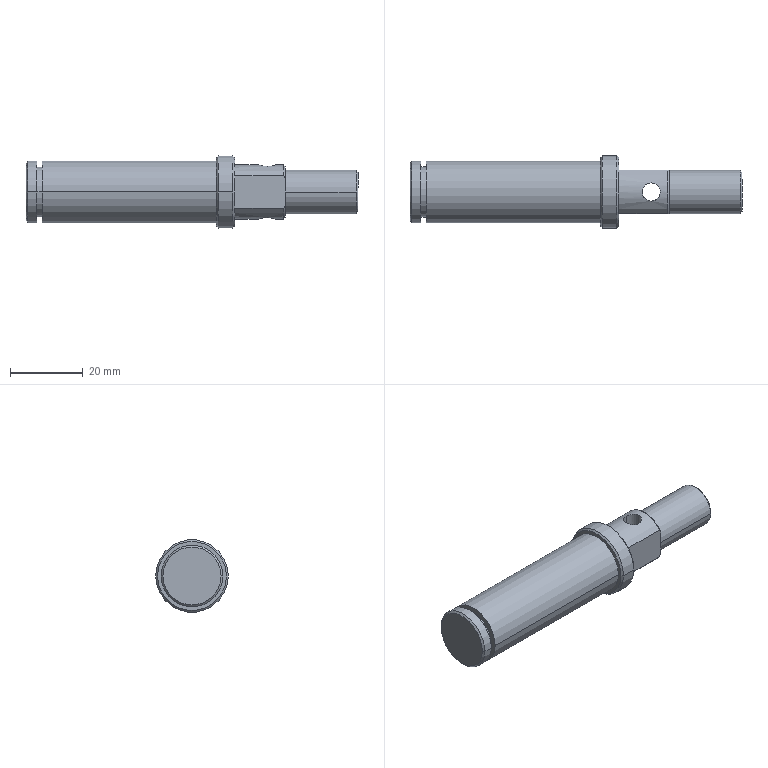Component | SolidWorks | CCD11-00TensioningAssembly-1_CCD11TensioningAxis-1 | 1 solid | 34 faces | box 91.5 x 20 x 20 mm | volume 17529 mm3 | cylinder 14 | cone 10 | plane 10 | commonest cylinder face diameters 17 x4 5 x2 12 x2 13.8 x2 20 x2 15 x2
STEP:
#1=CARTESIAN_POINT('',(-11.501,4.124,5.588));
#2=VERTEX_POINT('',#1);
#3=CARTESIAN_POINT('',(-11.501,4.321,5.588));
#4=VERTEX_POINT('',#3);
#5=CARTESIAN_POINT('',(-11.501,4.124,5.588));
#6=CARTESIAN_POINT('',(-11.507,4.124,5.588));
#7=CARTESIAN_POINT('',(-11.514,4.125,5.588));
#8=CARTESIAN_POINT('',(-11.526,4.127,5.587));
#9=CARTESIAN_POINT('',(-11.533,4.129,5.586));
#10=CARTESIAN_POINT('',(-11.545,4.134,5.584));
#11=CARTESIAN_POINT('',(-11.55,4.137,5.583));
#12=CARTESIAN_POINT('',(-11.561,4.144,5.581));
#13=CARTESIAN_POINT('',(-11.566,4.148,5.58));
#14=CARTESIAN_POINT('',(-11.579,4.162,5.577));
#15=CARTESIAN_POINT('',(-11.587,4.173,5.575));
#16=CARTESIAN_POINT('',(-11.594,4.191,5.573));
#17=CARTESIAN_POINT('',(-11.596,4.197,5.572));
#18=CARTESIAN_POINT('',(-11.599,4.21,5.571));
#19=CARTESIAN_POINT('',(-11.599,4.216,5.571));
#20=CARTESIAN_POINT('',(-11.599,4.229,5.571));
#21=CARTESIAN_POINT('',(-11.599,4.235,5.571));
#22=CARTESIAN_POINT('',(-11.596,4.248,5.572));
#23=CARTESIAN_POINT('',(-11.594,4.254,5.573));
#24=CARTESIAN_POINT('',(-11.589,4.266,5.574));
#25=CARTESIAN_POINT('',(-11.586,4.272,5.575));
#26=CARTESIAN_POINT('',(-11.579,4.283,5.577));
#27=CARTESIAN_POINT('',(-11.575,4.288,5.578));
#28=CARTESIAN_POINT('',(-11.566,4.297,5.58));
#29=CARTESIAN_POINT('',(-11.561,4.301,5.581));
#30=CARTESIAN_POINT('',(-11.55,4.308,5.583));
#31=CARTESIAN_POINT('',(-11.545,4.311,5.584));
#32=CARTESIAN_POINT('',(-11.533,4.316,5.586));
#33=CARTESIAN_POINT('',(-11.527,4.318,5.587));
#34=CARTESIAN_POINT('',(-11.514,4.32,5.588));
#35=CARTESIAN_POINT('',(-11.507,4.321,5.588));
#36=CARTESIAN_POINT('',(-11.501,4.321,5.588));
#37=B_SPLINE_CURVE_WITH_KNOTS('',3,(#5,#6,#7,#8,#9,#10,#11,#12,#13,#14,#15,#16,#17,#18,#19,#20,#21,#22,#23,#24,#25,#26,#27,#28,#29,#30,#31,#32,#33,#34,#35,#36),.UNSPECIFIED.,.F.,.F.,(4,2,2,2,2,2,2,2,2,2,2,2,2,2,2,4),(0.,0.000492,0.0009841,0.001476,0.001968,0.002952,0.003444,0.003936,0.004428,0.00492,0.005412,0.005905,0.006397,0.006889,0.007381,0.007873),.UNSPECIFIED.);
#38=EDGE_CURVE('',#2,#4,#37,.T.);
#39=ORIENTED_EDGE('',*,*,#38,.T.);
#40=CARTESIAN_POINT('',(-11.501,4.321,6.145));
#41=VERTEX_POINT('',#40);
#42=CARTESIAN_POINT('',(-11.501,4.321,6.161));
#43=DIRECTION('',(0.,0.,1.));
#44=VECTOR('',#43,39.37);
#45=LINE('',#42,#44);
#46=EDGE_CURVE('',#4,#41,#45,.T.);
#47=ORIENTED_EDGE('',*,*,#46,.T.);
#48=CARTESIAN_POINT('',(-11.501,4.124,6.145));
#49=VERTEX_POINT('',#48);
#50=CARTESIAN_POINT('',(-11.501,4.321,6.145));
#51=CARTESIAN_POINT('',(-11.507,4.321,6.145));
#52=CARTESIAN_POINT('',(-11.514,4.32,6.145));
#53=CARTESIAN_POINT('',(-11.527,4.318,6.146));
#54=CARTESIAN_POINT('',(-11.533,4.316,6.146));
#55=CARTESIAN_POINT('',(-11.545,4.311,6.148));
#56=CARTESIAN_POINT('',(-11.55,4.308,6.149));
#57=CARTESIAN_POINT('',(-11.561,4.301,6.151));
#58=CARTESIAN_POINT('',(-11.566,4.297,6.152));
#59=CARTESIAN_POINT('',(-11.58,4.283,6.155));
#60=CARTESIAN_POINT('',(-11.587,4.272,6.157));
#61=CARTESIAN_POINT('',(-11.594,4.254,6.16));
#62=CARTESIAN_POINT('',(-11.596,4.248,6.16));
#63=CARTESIAN_POINT('',(-11.599,4.236,6.161));
#64=CARTESIAN_POINT('',(-11.599,4.229,6.161));
#65=CARTESIAN_POINT('',(-11.599,4.216,6.161));
#66=CARTESIAN_POINT('',(-11.599,4.21,6.161));
#67=CARTESIAN_POINT('',(-11.596,4.197,6.16));
#68=CARTESIAN_POINT('',(-11.594,4.191,6.16));
#69=CARTESIAN_POINT('',(-11.587,4.173,6.157));
#70=CARTESIAN_POINT('',(-11.579,4.162,6.155));
#71=CARTESIAN_POINT('',(-11.566,4.148,6.152));
#72=CARTESIAN_POINT('',(-11.561,4.144,6.151));
#73=CARTESIAN_POINT('',(-11.55,4.137,6.149));
#74=CARTESIAN_POINT('',(-11.545,4.134,6.148));
#75=CARTESIAN_POINT('',(-11.533,4.129,6.146));
#76=CARTESIAN_POINT('',(-11.526,4.127,6.146));
#77=CARTESIAN_POINT('',(-11.514,4.125,6.145));
#78=CARTESIAN_POINT('',(-11.507,4.124,6.145));
#79=CARTESIAN_POINT('',(-11.501,4.124,6.145));
#80=B_SPLINE_CURVE_WITH_KNOTS('',3,(#50,#51,#52,#53,#54,#55,#56,#57,#58,#59,#60,#61,#62,#63,#64,#65,#66,#67,#68,#69,#70,#71,#72,#73,#74,#75,#76,#77,#78,#79),.UNSPECIFIED.,.F.,.F.,(4,2,2,2,2,2,2,2,2,2,2,2,2,2,4),(0.007873,0.008365,0.008857,0.009348,0.00984,0.01082,0.01132,0.01181,0.0123,0.01279,0.01378,0.01427,0.01476,0.01525,0.01574),.UNSPECIFIED.);
#81=EDGE_CURVE('',#41,#49,#80,.T.);
#82=ORIENTED_EDGE('',*,*,#81,.T.);
#83=CARTESIAN_POINT('',(-11.501,4.124,6.161));
#84=DIRECTION('',(0.,0.,1.));
#85=VECTOR('',#84,39.37);
#86=LINE('',#83,#85);
#87=EDGE_CURVE('',#2,#49,#86,.T.);
#88=ORIENTED_EDGE('',*,*,#87,.F.);
#89=EDGE_LOOP('',(#39,#47,#82,#88));
#90=FACE_OUTER_BOUND('',#89,.T.);
#91=CARTESIAN_POINT('',(-11.501,4.222,6.161));
#92=DIRECTION('',(0.,0.,1.));
#93=DIRECTION('',(0.,-1.,0.));
#94=AXIS2_PLACEMENT_3D('',#91,#92,#93);
#95=CYLINDRICAL_SURFACE('',#94,0.09843);
#96=ADVANCED_FACE('',(#90),#95,.F.);
#97=CARTESIAN_POINT('',(-11.855,4.597,5.866));
#98=VERTEX_POINT('',#97);
#99=CARTESIAN_POINT('',(-11.855,3.848,5.866));
#100=VERTEX_POINT('',#99);
#101=CARTESIAN_POINT('',(-11.855,4.222,5.866));
#102=DIRECTION('',(1.,0.,-0.));
#103=DIRECTION('',(-0.,1.,0.));
#104=AXIS2_PLACEMENT_3D('',#101,#102,#103);
#105=CIRCLE('',#104,0.374);
#106=EDGE_CURVE('',#98,#100,#105,.T.);
#107=ORIENTED_EDGE('',*,*,#106,.F.);
#108=CARTESIAN_POINT('',(-11.875,4.616,5.866));
#109=VERTEX_POINT('',#108);
#110=CARTESIAN_POINT('',(-11.875,4.616,5.866));
#111=DIRECTION('',(-0.7071,0.7071,0.));
#112=VECTOR('',#111,39.37);
#113=LINE('',#110,#112);
#114=EDGE_CURVE('',#98,#109,#113,.T.);
#115=ORIENTED_EDGE('',*,*,#114,.T.);
#116=CARTESIAN_POINT('',(-11.875,3.829,5.866));
#117=VERTEX_POINT('',#116);
#118=CARTESIAN_POINT('',(-11.875,4.222,5.866));
#119=DIRECTION('',(-1.,-0.,0.));
#120=DIRECTION('',(-0.,1.,-0.));
#121=AXIS2_PLACEMENT_3D('',#118,#119,#120);
#122=CIRCLE('',#121,0.3937);
#123=EDGE_CURVE('',#117,#109,#122,.T.);
#124=ORIENTED_EDGE('',*,*,#123,.F.);
#125=CARTESIAN_POINT('',(-11.875,3.829,5.866));
#126=DIRECTION('',(-0.7071,-0.7071,0.));
#127=VECTOR('',#126,39.37);
#128=LINE('',#125,#127);
#129=EDGE_CURVE('',#100,#117,#128,.T.);
#130=ORIENTED_EDGE('',*,*,#129,.F.);
#131=EDGE_LOOP('',(#107,#115,#124,#130));
#132=FACE_OUTER_BOUND('',#131,.T.);
#133=CARTESIAN_POINT('',(-11.875,4.222,5.866));
#134=DIRECTION('',(-1.,-0.,0.));
#135=DIRECTION('',(0.,-1.,0.));
#136=AXIS2_PLACEMENT_3D('',#133,#134,#135);
#137=CONICAL_SURFACE('',#136,0.3937,0.7854);
#138=ADVANCED_FACE('',(#132),#137,.T.);
#139=CARTESIAN_POINT('',(-10.517,4.439,5.866));
#140=VERTEX_POINT('',#139);
#141=CARTESIAN_POINT('',(-10.517,4.006,5.866));
#142=VERTEX_POINT('',#141);
#143=CARTESIAN_POINT('',(-10.517,4.222,5.866));
#144=DIRECTION('',(1.,0.,-0.));
#145=DIRECTION('',(0.,-1.,0.));
#146=AXIS2_PLACEMENT_3D('',#143,#144,#145);
#147=CIRCLE('',#146,0.2165);
#148=EDGE_CURVE('',#140,#142,#147,.T.);
#149=ORIENTED_EDGE('',*,*,#148,.F.);
#150=CARTESIAN_POINT('',(-10.536,4.459,5.866));
#151=VERTEX_POINT('',#150);
#152=CARTESIAN_POINT('',(-10.536,4.459,5.866));
#153=DIRECTION('',(-0.7071,0.7071,0.));
#154=VECTOR('',#153,39.37);
#155=LINE('',#152,#154);
#156=EDGE_CURVE('',#140,#151,#155,.T.);
#157=ORIENTED_EDGE('',*,*,#156,.T.);
#158=CARTESIAN_POINT('',(-10.536,3.986,5.866));
#159=VERTEX_POINT('',#158);
#160=CARTESIAN_POINT('',(-10.536,4.222,5.866));
#161=DIRECTION('',(-1.,-0.,0.));
#162=DIRECTION('',(0.,-1.,0.));
#163=AXIS2_PLACEMENT_3D('',#160,#161,#162);
#164=CIRCLE('',#163,0.2362);
#165=EDGE_CURVE('',#159,#151,#164,.T.);
#166=ORIENTED_EDGE('',*,*,#165,.F.);
#167=CARTESIAN_POINT('',(-10.536,3.986,5.866));
#168=DIRECTION('',(-0.7071,-0.7071,0.));
#169=VECTOR('',#168,39.37);
#170=LINE('',#167,#169);
#171=EDGE_CURVE('',#142,#159,#170,.T.);
#172=ORIENTED_EDGE('',*,*,#171,.F.);
#173=EDGE_LOOP('',(#149,#157,#166,#172));
#174=FACE_OUTER_BOUND('',#173,.T.);
#175=CARTESIAN_POINT('',(-10.536,4.222,5.866));
#176=DIRECTION('',(-1.,-0.,0.));
#177=DIRECTION('',(0.,-1.,0.));
#178=AXIS2_PLACEMENT_3D('',#175,#176,#177);
#179=CONICAL_SURFACE('',#178,0.2362,0.7854);
#180=ADVANCED_FACE('',(#174),#179,.T.);
#181=CARTESIAN_POINT('',(-12.052,3.848,5.866));
#182=VERTEX_POINT('',#181);
#183=CARTESIAN_POINT('',(-12.052,4.597,5.866));
#184=VERTEX_POINT('',#183);
#185=CARTESIAN_POINT('',(-12.052,4.222,5.866));
#186=DIRECTION('',(-1.,-0.,0.));
#187=DIRECTION('',(-0.,1.,0.));
#188=AXIS2_PLACEMENT_3D('',#185,#186,#187);
#189=CIRCLE('',#188,0.374);
#190=EDGE_CURVE('',#182,#184,#189,.T.);
#191=ORIENTED_EDGE('',*,*,#190,.F.);
#192=CARTESIAN_POINT('',(-12.032,3.829,5.866));
#193=VERTEX_POINT('',#192);
#194=CARTESIAN_POINT('',(-12.052,3.848,5.866));
#195=DIRECTION('',(0.7071,-0.7071,-0.));
#196=VECTOR('',#195,39.37);
#197=LINE('',#194,#196);
#198=EDGE_CURVE('',#182,#193,#197,.T.);
#199=ORIENTED_EDGE('',*,*,#198,.T.);
#200=CARTESIAN_POINT('',(-12.032,4.616,5.866));
#201=VERTEX_POINT('',#200);
#202=CARTESIAN_POINT('',(-12.032,4.222,5.866));
#203=DIRECTION('',(1.,0.,-0.));
#204=DIRECTION('',(-0.,1.,0.));
#205=AXIS2_PLACEMENT_3D('',#202,#203,#204);
#206=CIRCLE('',#205,0.3937);
#207=EDGE_CURVE('',#201,#193,#206,.T.);
#208=ORIENTED_EDGE('',*,*,#207,.F.);
#209=CARTESIAN_POINT('',(-12.052,4.597,5.866));
#210=DIRECTION('',(0.7071,0.7071,-0.));
#211=VECTOR('',#210,39.37);
#212=LINE('',#209,#211);
#213=EDGE_CURVE('',#184,#201,#212,.T.);
#214=ORIENTED_EDGE('',*,*,#213,.F.);
#215=EDGE_LOOP('',(#191,#199,#208,#214));
#216=FACE_OUTER_BOUND('',#215,.T.);
#217=CARTESIAN_POINT('',(-12.052,4.222,5.866));
#218=DIRECTION('',(1.,0.,-0.));
#219=DIRECTION('',(-0.,1.,0.));
#220=AXIS2_PLACEMENT_3D('',#217,#218,#219);
#221=CONICAL_SURFACE('',#220,0.374,0.7854);
#222=ADVANCED_FACE('',(#216),#221,.T.);
#223=CARTESIAN_POINT('',(-14.119,3.908,5.866));
#224=VERTEX_POINT('',#223);
#225=CARTESIAN_POINT('',(-14.119,4.537,5.866));
#226=VERTEX_POINT('',#225);
#227=CARTESIAN_POINT('',(-14.119,4.222,5.866));
#228=DIRECTION('',(-1.,-0.,0.));
#229=DIRECTION('',(-0.,1.,0.));
#230=AXIS2_PLACEMENT_3D('',#227,#228,#229);
#231=CIRCLE('',#230,0.315);
#232=EDGE_CURVE('',#224,#226,#231,.T.);
#233=ORIENTED_EDGE('',*,*,#232,.F.);
#234=CARTESIAN_POINT('',(-14.099,3.888,5.866));
#235=VERTEX_POINT('',#234);
#236=CARTESIAN_POINT('',(-14.119,3.908,5.866));
#237=DIRECTION('',(0.7071,-0.7071,-0.));
#238=VECTOR('',#237,39.37);
#239=LINE('',#236,#238);
#240=EDGE_CURVE('',#224,#235,#239,.T.);
#241=ORIENTED_EDGE('',*,*,#240,.T.);
#242=CARTESIAN_POINT('',(-14.099,4.557,5.866));
#243=VERTEX_POINT('',#242);
#244=CARTESIAN_POINT('',(-14.099,4.222,5.866));
#245=DIRECTION('',(1.,0.,-0.));
#246=DIRECTION('',(-0.,1.,0.));
#247=AXIS2_PLACEMENT_3D('',#244,#245,#246);
#248=CIRCLE('',#247,0.3346);
#249=EDGE_CURVE('',#243,#235,#248,.T.);
#250=ORIENTED_EDGE('',*,*,#249,.F.);
#251=CARTESIAN_POINT('',(-14.119,4.537,5.866));
#252=DIRECTION('',(0.7071,0.7071,-0.));
#253=VECTOR('',#252,39.37);
#254=LINE('',#251,#253);
#255=EDGE_CURVE('',#226,#243,#254,.T.);
#256=ORIENTED_EDGE('',*,*,#255,.F.);
#257=EDGE_LOOP('',(#233,#241,#250,#256));
#258=FACE_OUTER_BOUND('',#257,.T.);
#259=CARTESIAN_POINT('',(-14.119,4.222,5.866));
#260=DIRECTION('',(1.,0.,-0.));
#261=DIRECTION('',(-0.,1.,0.));
#262=AXIS2_PLACEMENT_3D('',#259,#260,#261);
#263=CONICAL_SURFACE('',#262,0.315,0.7854);
#264=ADVANCED_FACE('',(#258),#263,.T.);
#265=ORIENTED_EDGE('',*,*,#165,.T.);
#266=CARTESIAN_POINT('',(-11.304,4.459,5.866));
#267=VERTEX_POINT('',#266);
#268=CARTESIAN_POINT('',(-17.357,4.459,5.866));
#269=DIRECTION('',(-1.,-0.,0.));
#270=VECTOR('',#269,39.37);
#271=LINE('',#268,#270);
#272=EDGE_CURVE('',#151,#267,#271,.T.);
#273=ORIENTED_EDGE('',*,*,#272,.T.);
#274=CARTESIAN_POINT('',(-11.304,3.986,5.866));
#275=VERTEX_POINT('',#274);
#276=CARTESIAN_POINT('',(-11.304,4.222,5.866));
#277=DIRECTION('',(-1.,-0.,0.));
#278=DIRECTION('',(0.,-1.,0.));
#279=AXIS2_PLACEMENT_3D('',#276,#277,#278);
#280=CIRCLE('',#279,0.2362);
#281=EDGE_CURVE('',#275,#267,#280,.T.);
#282=ORIENTED_EDGE('',*,*,#281,.F.);
#283=CARTESIAN_POINT('',(-17.357,3.986,5.866));
#284=DIRECTION('',(-1.,-0.,0.));
#285=VECTOR('',#284,39.37);
#286=LINE('',#283,#285);
#287=EDGE_CURVE('',#159,#275,#286,.T.);
#288=ORIENTED_EDGE('',*,*,#287,.F.);
#289=EDGE_LOOP('',(#265,#273,#282,#288));
#290=FACE_OUTER_BOUND('',#289,.T.);
#291=CARTESIAN_POINT('',(-17.357,4.222,5.866));
#292=DIRECTION('',(-1.,-0.,0.));
#293=DIRECTION('',(0.,-1.,0.));
#294=AXIS2_PLACEMENT_3D('',#291,#292,#293);
#295=CYLINDRICAL_SURFACE('',#294,0.2362);
#296=ADVANCED_FACE('',(#290),#295,.T.);
#297=CARTESIAN_POINT('',(-12.052,3.888,5.866));
#298=VERTEX_POINT('',#297);
#299=CARTESIAN_POINT('',(-12.052,4.557,5.866));
#300=VERTEX_POINT('',#299);
#301=CARTESIAN_POINT('',(-12.052,4.222,5.866));
#302=DIRECTION('',(-1.,-0.,0.));
#303=DIRECTION('',(0.,-1.,0.));
#304=AXIS2_PLACEMENT_3D('',#301,#302,#303);
#305=CIRCLE('',#304,0.3346);
#306=EDGE_CURVE('',#298,#300,#305,.T.);
#307=ORIENTED_EDGE('',*,*,#306,.T.);
#308=CARTESIAN_POINT('',(-13.942,4.557,5.866));
#309=VERTEX_POINT('',#308);
#310=CARTESIAN_POINT('',(-17.357,4.557,5.866));
#311=DIRECTION('',(-1.,-0.,0.));
#312=VECTOR('',#311,39.37);
#313=LINE('',#310,#312);
#314=EDGE_CURVE('',#300,#309,#313,.T.);
#315=ORIENTED_EDGE('',*,*,#314,.T.);
#316=CARTESIAN_POINT('',(-13.942,3.888,5.866));
#317=VERTEX_POINT('',#316);
#318=CARTESIAN_POINT('',(-13.942,4.222,5.866));
#319=DIRECTION('',(-1.,-0.,0.));
#320=DIRECTION('',(0.,-1.,0.));
#321=AXIS2_PLACEMENT_3D('',#318,#319,#320);
#322=CIRCLE('',#321,0.3346);
#323=EDGE_CURVE('',#317,#309,#322,.T.);
#324=ORIENTED_EDGE('',*,*,#323,.F.);
#325=CARTESIAN_POINT('',(-17.357,3.888,5.866));
#326=DIRECTION('',(-1.,-0.,0.));
#327=VECTOR('',#326,39.37);
#328=LINE('',#325,#327);
#329=EDGE_CURVE('',#298,#317,#328,.T.);
#330=ORIENTED_EDGE('',*,*,#329,.F.);
#331=EDGE_LOOP('',(#307,#315,#324,#330));
#332=FACE_OUTER_BOUND('',#331,.T.);
#333=CARTESIAN_POINT('',(-17.357,4.222,5.866));
#334=DIRECTION('',(-1.,-0.,0.));
#335=DIRECTION('',(0.,-1.,0.));
#336=AXIS2_PLACEMENT_3D('',#333,#334,#335);
#337=CYLINDRICAL_SURFACE('',#336,0.3346);
#338=ADVANCED_FACE('',(#332),#337,.T.);
#339=CARTESIAN_POINT('',(-13.942,3.951,5.866));
#340=VERTEX_POINT('',#339);
#341=CARTESIAN_POINT('',(-13.942,4.494,5.866));
#342=VERTEX_POINT('',#341);
#343=CARTESIAN_POINT('',(-13.942,4.222,5.866));
#344=DIRECTION('',(-1.,-0.,0.));
#345=DIRECTION('',(0.,-1.,0.));
#346=AXIS2_PLACEMENT_3D('',#343,#344,#345);
#347=CIRCLE('',#346,0.2717);
#348=EDGE_CURVE('',#340,#342,#347,.T.);
#349=ORIENTED_EDGE('',*,*,#348,.T.);
#350=CARTESIAN_POINT('',(-14.001,4.494,5.866));
#351=VERTEX_POINT('',#350);
#352=CARTESIAN_POINT('',(-17.357,4.494,5.866));
#353=DIRECTION('',(-1.,-0.,0.));
#354=VECTOR('',#353,39.37);
#355=LINE('',#352,#354);
#356=EDGE_CURVE('',#342,#351,#355,.T.);
#357=ORIENTED_EDGE('',*,*,#356,.T.);
#358=CARTESIAN_POINT('',(-14.001,3.951,5.866));
#359=VERTEX_POINT('',#358);
#360=CARTESIAN_POINT('',(-14.001,4.222,5.866));
#361=DIRECTION('',(-1.,-0.,0.));
#362=DIRECTION('',(0.,-1.,0.));
#363=AXIS2_PLACEMENT_3D('',#360,#361,#362);
#364=CIRCLE('',#363,0.2717);
#365=EDGE_CURVE('',#359,#351,#364,.T.);
#366=ORIENTED_EDGE('',*,*,#365,.F.);
#367=CARTESIAN_POINT('',(-17.357,3.951,5.866));
#368=DIRECTION('',(-1.,-0.,0.));
#369=VECTOR('',#368,39.37);
#370=LINE('',#367,#369);
#371=EDGE_CURVE('',#340,#359,#370,.T.);
#372=ORIENTED_EDGE('',*,*,#371,.F.);
#373=EDGE_LOOP('',(#349,#357,#366,#372));
#374=FACE_OUTER_BOUND('',#373,.T.);
#375=CARTESIAN_POINT('',(-17.357,4.222,5.866));
#376=DIRECTION('',(-1.,-0.,0.));
#377=DIRECTION('',(0.,-1.,0.));
#378=AXIS2_PLACEMENT_3D('',#375,#376,#377);
#379=CYLINDRICAL_SURFACE('',#378,0.2717);
#380=ADVANCED_FACE('',(#374),#379,.T.);
#381=CARTESIAN_POINT('',(-14.001,3.888,5.866));
#382=VERTEX_POINT('',#381);
#383=CARTESIAN_POINT('',(-14.001,4.557,5.866));
#384=VERTEX_POINT('',#383);
#385=CARTESIAN_POINT('',(-14.001,4.222,5.866));
#386=DIRECTION('',(-1.,-0.,0.));
#387=DIRECTION('',(0.,-1.,0.));
#388=AXIS2_PLACEMENT_3D('',#385,#386,#387);
#389=CIRCLE('',#388,0.3346);
#390=EDGE_CURVE('',#382,#384,#389,.T.);
#391=ORIENTED_EDGE('',*,*,#390,.T.);
#392=CARTESIAN_POINT('',(-17.357,4.557,5.866));
#393=DIRECTION('',(-1.,-0.,0.));
#394=VECTOR('',#393,39.37);
#395=LINE('',#392,#394);
#396=EDGE_CURVE('',#384,#243,#395,.T.);
#397=ORIENTED_EDGE('',*,*,#396,.T.);
#398=ORIENTED_EDGE('',*,*,#249,.T.);
#399=CARTESIAN_POINT('',(-17.357,3.888,5.866));
#400=DIRECTION('',(-1.,-0.,0.));
#401=VECTOR('',#400,39.37);
#402=LINE('',#399,#401);
#403=EDGE_CURVE('',#382,#235,#402,.T.);
#404=ORIENTED_EDGE('',*,*,#403,.F.);
#405=EDGE_LOOP('',(#391,#397,#398,#404));
#406=FACE_OUTER_BOUND('',#405,.T.);
#407=CARTESIAN_POINT('',(-17.357,4.222,5.866));
#408=DIRECTION('',(-1.,-0.,0.));
#409=DIRECTION('',(0.,-1.,0.));
#410=AXIS2_PLACEMENT_3D('',#407,#408,#409);
#411=CYLINDRICAL_SURFACE('',#410,0.3346);
#412=ADVANCED_FACE('',(#406),#411,.T.);
#413=ORIENTED_EDGE('',*,*,#123,.T.);
#414=CARTESIAN_POINT('',(-17.357,4.616,5.866));
#415=DIRECTION('',(-1.,-0.,0.));
#416=VECTOR('',#415,39.37);
#417=LINE('',#414,#416);
#418=EDGE_CURVE('',#109,#201,#417,.T.);
#419=ORIENTED_EDGE('',*,*,#418,.T.);
#420=ORIENTED_EDGE('',*,*,#207,.T.);
#421=CARTESIAN_POINT('',(-17.357,3.829,5.866));
#422=DIRECTION('',(-1.,-0.,0.));
#423=VECTOR('',#422,39.37);
#424=LINE('',#421,#423);
#425=EDGE_CURVE('',#117,#193,#424,.T.);
#426=ORIENTED_EDGE('',*,*,#425,.F.);
#427=EDGE_LOOP('',(#413,#419,#420,#426));
#428=FACE_OUTER_BOUND('',#427,.T.);
#429=CARTESIAN_POINT('',(-17.357,4.222,5.866));
#430=DIRECTION('',(-1.,-0.,0.));
#431=DIRECTION('',(0.,-1.,0.));
#432=AXIS2_PLACEMENT_3D('',#429,#430,#431);
#433=CYLINDRICAL_SURFACE('',#432,0.3937);
#434=ADVANCED_FACE('',(#428),#433,.T.);
#435=CARTESIAN_POINT('',(-11.304,4.459,6.008));
#436=VERTEX_POINT('',#435);
#437=CARTESIAN_POINT('',(-11.304,4.459,6.259));
#438=DIRECTION('',(-0.,0.,-1.));
#439=VECTOR('',#438,39.37);
#440=LINE('',#437,#439);
#441=EDGE_CURVE('',#436,#267,#440,.T.);
#442=ORIENTED_EDGE('',*,*,#441,.F.);
#443=CARTESIAN_POINT('',(-11.304,3.986,6.008));
#444=VERTEX_POINT('',#443);
#445=CARTESIAN_POINT('',(-11.304,4.222,5.866));
#446=DIRECTION('',(1.,0.,-0.));
#447=DIRECTION('',(0.,-1.,-0.));
#448=AXIS2_PLACEMENT_3D('',#445,#446,#447);
#449=CIRCLE('',#448,0.2756);
#450=EDGE_CURVE('',#436,#444,#449,.T.);
#451=ORIENTED_EDGE('',*,*,#450,.T.);
#452=CARTESIAN_POINT('',(-11.304,3.986,6.261));
#453=DIRECTION('',(0.,-0.,1.));
#454=VECTOR('',#453,39.37);
#455=LINE('',#452,#454);
#456=EDGE_CURVE('',#275,#444,#455,.T.);
#457=ORIENTED_EDGE('',*,*,#456,.F.);
#458=ORIENTED_EDGE('',*,*,#281,.T.);
#459=EDGE_LOOP('',(#442,#451,#457,#458));
#460=FACE_OUTER_BOUND('',#459,.T.);
#461=CARTESIAN_POINT('',(-11.304,4.222,6.26));
#462=DIRECTION('',(-1.,-0.,0.));
#463=DIRECTION('',(0.,-1.,0.));
#464=AXIS2_PLACEMENT_3D('',#461,#462,#463);
#465=PLANE('',#464);
#466=ADVANCED_FACE('',(#460),#465,.F.);
#467=ORIENTED_EDGE('',*,*,#418,.F.);
#468=CARTESIAN_POINT('',(-11.875,4.222,5.866));
#469=DIRECTION('',(-1.,-0.,0.));
#470=DIRECTION('',(-0.,1.,0.));
#471=AXIS2_PLACEMENT_3D('',#468,#469,#470);
#472=CIRCLE('',#471,0.3937);
#473=EDGE_CURVE('',#109,#117,#472,.T.);
#474=ORIENTED_EDGE('',*,*,#473,.T.);
#475=ORIENTED_EDGE('',*,*,#425,.T.);
#476=CARTESIAN_POINT('',(-12.032,4.222,5.866));
#477=DIRECTION('',(1.,0.,-0.));
#478=DIRECTION('',(-0.,1.,0.));
#479=AXIS2_PLACEMENT_3D('',#476,#477,#478);
#480=CIRCLE('',#479,0.3937);
#481=EDGE_CURVE('',#193,#201,#480,.T.);
#482=ORIENTED_EDGE('',*,*,#481,.T.);
#483=EDGE_LOOP('',(#467,#474,#475,#482));
#484=FACE_OUTER_BOUND('',#483,.T.);
#485=CARTESIAN_POINT('',(-17.357,4.222,5.866));
#486=DIRECTION('',(-1.,-0.,0.));
#487=DIRECTION('',(0.,-1.,0.));
#488=AXIS2_PLACEMENT_3D('',#485,#486,#487);
#489=CYLINDRICAL_SURFACE('',#488,0.3937);
#490=ADVANCED_FACE('',(#484),#489,.T.);
#491=CARTESIAN_POINT('',(-11.304,3.986,5.724));
#492=VERTEX_POINT('',#491);
#493=CARTESIAN_POINT('',(-11.304,3.986,6.261));
#494=DIRECTION('',(0.,-0.,1.));
#495=VECTOR('',#494,39.37);
#496=LINE('',#493,#495);
#497=EDGE_CURVE('',#492,#275,#496,.T.);
#498=ORIENTED_EDGE('',*,*,#497,.F.);
#499=CARTESIAN_POINT('',(-11.304,4.459,5.724));
#500=VERTEX_POINT('',#499);
#501=CARTESIAN_POINT('',(-11.304,4.222,5.866));
#502=DIRECTION('',(1.,0.,-0.));
#503=DIRECTION('',(0.,-1.,0.));
#504=AXIS2_PLACEMENT_3D('',#501,#502,#503);
#505=CIRCLE('',#504,0.2756);
#506=EDGE_CURVE('',#492,#500,#505,.T.);
#507=ORIENTED_EDGE('',*,*,#506,.T.);
#508=CARTESIAN_POINT('',(-11.304,4.459,6.259));
#509=DIRECTION('',(-0.,0.,-1.));
#510=VECTOR('',#509,39.37);
#511=LINE('',#508,#510);
#512=EDGE_CURVE('',#267,#500,#511,.T.);
#513=ORIENTED_EDGE('',*,*,#512,.F.);
#514=CARTESIAN_POINT('',(-11.304,4.222,5.866));
#515=DIRECTION('',(-1.,-0.,0.));
#516=DIRECTION('',(0.,-1.,0.));
#517=AXIS2_PLACEMENT_3D('',#514,#515,#516);
#518=CIRCLE('',#517,0.2362);
#519=EDGE_CURVE('',#267,#275,#518,.T.);
#520=ORIENTED_EDGE('',*,*,#519,.T.);
#521=EDGE_LOOP('',(#498,#507,#513,#520));
#522=FACE_OUTER_BOUND('',#521,.T.);
#523=CARTESIAN_POINT('',(-11.304,4.222,6.26));
#524=DIRECTION('',(-1.,-0.,0.));
#525=DIRECTION('',(0.,-1.,0.));
#526=AXIS2_PLACEMENT_3D('',#523,#524,#525);
#527=PLANE('',#526);
#528=ADVANCED_FACE('',(#522),#527,.F.);
#529=CARTESIAN_POINT('',(-11.324,4.459,6.043));
#530=VERTEX_POINT('',#529);
#531=CARTESIAN_POINT('',(-11.855,4.459,6.043));
#532=VERTEX_POINT('',#531);
#533=CARTESIAN_POINT('',(-11.855,4.459,6.043));
#534=DIRECTION('',(-1.,-0.,0.));
#535=VECTOR('',#534,39.37);
#536=LINE('',#533,#535);
#537=EDGE_CURVE('',#530,#532,#536,.T.);
#538=ORIENTED_EDGE('',*,*,#537,.F.);
#539=CARTESIAN_POINT('',(-11.324,4.459,6.043));
#540=CARTESIAN_POINT('',(-11.317,4.459,6.032));
#541=CARTESIAN_POINT('',(-11.31,4.459,6.02));
#542=CARTESIAN_POINT('',(-11.304,4.459,6.008));
#543=B_SPLINE_CURVE_WITH_KNOTS('',3,(#539,#540,#541,#542),.UNSPECIFIED.,.F.,.F.,(4,4),(0.,0.001025),.UNSPECIFIED.);
#544=EDGE_CURVE('',#530,#436,#543,.T.);
#545=ORIENTED_EDGE('',*,*,#544,.T.);
#546=ORIENTED_EDGE('',*,*,#441,.T.);
#547=ORIENTED_EDGE('',*,*,#512,.T.);
#548=CARTESIAN_POINT('',(-11.324,4.459,5.689));
#549=VERTEX_POINT('',#548);
#550=CARTESIAN_POINT('',(-11.304,4.459,5.724));
#551=CARTESIAN_POINT('',(-11.31,4.459,5.712));
#552=CARTESIAN_POINT('',(-11.317,4.459,5.701));
#553=CARTESIAN_POINT('',(-11.324,4.459,5.689));
#554=B_SPLINE_CURVE_WITH_KNOTS('',3,(#550,#551,#552,#553),.UNSPECIFIED.,.F.,.F.,(4,4),(0.,0.001025),.UNSPECIFIED.);
#555=EDGE_CURVE('',#500,#549,#554,.T.);
#556=ORIENTED_EDGE('',*,*,#555,.T.);
#557=CARTESIAN_POINT('',(-11.855,4.459,5.689));
#558=VERTEX_POINT('',#557);
#559=CARTESIAN_POINT('',(-11.855,4.459,5.689));
#560=DIRECTION('',(1.,0.,-0.));
#561=VECTOR('',#560,39.37);
#562=LINE('',#559,#561);
#563=EDGE_CURVE('',#558,#549,#562,.T.);
#564=ORIENTED_EDGE('',*,*,#563,.F.);
#565=CARTESIAN_POINT('',(-11.855,4.459,6.259));
#566=DIRECTION('',(-0.,0.,-1.));
#567=VECTOR('',#566,39.37);
#568=LINE('',#565,#567);
#569=EDGE_CURVE('',#532,#558,#568,.T.);
#570=ORIENTED_EDGE('',*,*,#569,.F.);
#571=EDGE_LOOP('',(#538,#545,#546,#547,#556,#564,#570));
#572=FACE_OUTER_BOUND('',#571,.T.);
#573=CARTESIAN_POINT('',(-11.855,4.459,6.259));
#574=DIRECTION('',(0.,-1.,-0.));
#575=DIRECTION('',(-0.,0.,-1.));
#576=AXIS2_PLACEMENT_3D('',#573,#574,#575);
#577=PLANE('',#576);
#578=ADVANCED_FACE('',(#572),#577,.F.);
#579=ORIENTED_EDGE('',*,*,#456,.T.);
#580=CARTESIAN_POINT('',(-11.324,3.986,6.043));
#581=VERTEX_POINT('',#580);
#582=CARTESIAN_POINT('',(-11.304,3.986,6.008));
#583=CARTESIAN_POINT('',(-11.31,3.986,6.02));
#584=CARTESIAN_POINT('',(-11.317,3.986,6.032));
#585=CARTESIAN_POINT('',(-11.324,3.986,6.043));
#586=B_SPLINE_CURVE_WITH_KNOTS('',3,(#582,#583,#584,#585),.UNSPECIFIED.,.F.,.F.,(4,4),(0.,0.001025),.UNSPECIFIED.);
#587=EDGE_CURVE('',#444,#581,#586,.T.);
#588=ORIENTED_EDGE('',*,*,#587,.T.);
#589=CARTESIAN_POINT('',(-11.855,3.986,6.043));
#590=VERTEX_POINT('',#589);
#591=CARTESIAN_POINT('',(-11.855,3.986,6.043));
#592=DIRECTION('',(1.,0.,-0.));
#593=VECTOR('',#592,39.37);
#594=LINE('',#591,#593);
#595=EDGE_CURVE('',#590,#581,#594,.T.);
#596=ORIENTED_EDGE('',*,*,#595,.F.);
#597=CARTESIAN_POINT('',(-11.855,3.986,5.689));
#598=VERTEX_POINT('',#597);
#599=CARTESIAN_POINT('',(-11.855,3.986,6.261));
#600=DIRECTION('',(0.,-0.,1.));
#601=VECTOR('',#600,39.37);
#602=LINE('',#599,#601);
#603=EDGE_CURVE('',#598,#590,#602,.T.);
#604=ORIENTED_EDGE('',*,*,#603,.F.);
#605=CARTESIAN_POINT('',(-11.324,3.986,5.689));
#606=VERTEX_POINT('',#605);
#607=CARTESIAN_POINT('',(-11.855,3.986,5.689));
#608=DIRECTION('',(-1.,-0.,0.));
#609=VECTOR('',#608,39.37);
#610=LINE('',#607,#609);
#611=EDGE_CURVE('',#606,#598,#610,.T.);
#612=ORIENTED_EDGE('',*,*,#611,.F.);
#613=CARTESIAN_POINT('',(-11.324,3.986,5.689));
#614=CARTESIAN_POINT('',(-11.317,3.986,5.701));
#615=CARTESIAN_POINT('',(-11.31,3.986,5.712));
#616=CARTESIAN_POINT('',(-11.304,3.986,5.724));
#617=B_SPLINE_CURVE_WITH_KNOTS('',3,(#613,#614,#615,#616),.UNSPECIFIED.,.F.,.F.,(4,4),(0.,0.001025),.UNSPECIFIED.);
#618=EDGE_CURVE('',#606,#492,#617,.T.);
#619=ORIENTED_EDGE('',*,*,#618,.T.);
#620=ORIENTED_EDGE('',*,*,#497,.T.);
#621=EDGE_LOOP('',(#579,#588,#596,#604,#612,#619,#620));
#622=FACE_OUTER_BOUND('',#621,.T.);
#623=CARTESIAN_POINT('',(-11.855,3.986,6.261));
#624=DIRECTION('',(-0.,1.,0.));
#625=DIRECTION('',(0.,-0.,1.));
#626=AXIS2_PLACEMENT_3D('',#623,#624,#625);
#627=PLANE('',#626);
#628=ADVANCED_FACE('',(#622),#627,.F.);
#629=CARTESIAN_POINT('',(-14.119,4.222,5.866));
#630=DIRECTION('',(-1.,-0.,0.));
#631=DIRECTION('',(-0.,1.,0.));
#632=AXIS2_PLACEMENT_3D('',#629,#630,#631);
#633=CIRCLE('',#632,0.315);
#634=EDGE_CURVE('',#226,#224,#633,.T.);
#635=ORIENTED_EDGE('',*,*,#634,.T.);
#636=ORIENTED_EDGE('',*,*,#232,.T.);
#637=EDGE_LOOP('',(#635,#636));
#638=FACE_OUTER_BOUND('',#637,.T.);
#639=CARTESIAN_POINT('',(-14.119,4.222,5.866));
#640=DIRECTION('',(1.,0.,-0.));
#641=DIRECTION('',(-0.,1.,-0.));
#642=AXIS2_PLACEMENT_3D('',#639,#640,#641);
#643=PLANE('',#642);
#644=ADVANCED_FACE('',(#638),#643,.F.);
#645=ORIENTED_EDGE('',*,*,#396,.F.);
#646=CARTESIAN_POINT('',(-14.001,4.222,5.866));
#647=DIRECTION('',(-1.,-0.,0.));
#648=DIRECTION('',(0.,-1.,0.));
#649=AXIS2_PLACEMENT_3D('',#646,#647,#648);
#650=CIRCLE('',#649,0.3346);
#651=EDGE_CURVE('',#384,#382,#650,.T.);
#652=ORIENTED_EDGE('',*,*,#651,.T.);
#653=ORIENTED_EDGE('',*,*,#403,.T.);
#654=CARTESIAN_POINT('',(-14.099,4.222,5.866));
#655=DIRECTION('',(1.,0.,-0.));
#656=DIRECTION('',(-0.,1.,0.));
#657=AXIS2_PLACEMENT_3D('',#654,#655,#656);
#658=CIRCLE('',#657,0.3346);
#659=EDGE_CURVE('',#235,#243,#658,.T.);
#660=ORIENTED_EDGE('',*,*,#659,.T.);
#661=EDGE_LOOP('',(#645,#652,#653,#660));
#662=FACE_OUTER_BOUND('',#661,.T.);
#663=CARTESIAN_POINT('',(-17.357,4.222,5.866));
#664=DIRECTION('',(-1.,-0.,0.));
#665=DIRECTION('',(0.,-1.,0.));
#666=AXIS2_PLACEMENT_3D('',#663,#664,#665);
#667=CYLINDRICAL_SURFACE('',#666,0.3346);
#668=ADVANCED_FACE('',(#662),#667,.T.);
#669=ORIENTED_EDGE('',*,*,#390,.F.);
#670=ORIENTED_EDGE('',*,*,#651,.F.);
#671=EDGE_LOOP('',(#669,#670));
#672=FACE_OUTER_BOUND('',#671,.T.);
#673=ORIENTED_EDGE('',*,*,#365,.T.);
#674=CARTESIAN_POINT('',(-14.001,4.222,5.866));
#675=DIRECTION('',(-1.,-0.,0.));
#676=DIRECTION('',(0.,-1.,0.));
#677=AXIS2_PLACEMENT_3D('',#674,#675,#676);
#678=CIRCLE('',#677,0.2717);
#679=EDGE_CURVE('',#351,#359,#678,.T.);
#680=ORIENTED_EDGE('',*,*,#679,.T.);
#681=EDGE_LOOP('',(#673,#680));
#682=FACE_BOUND('',#681,.T.);
#683=CARTESIAN_POINT('',(-14.001,4.222,6.201));
#684=DIRECTION('',(-1.,-0.,0.));
#685=DIRECTION('',(0.,-1.,0.));
#686=AXIS2_PLACEMENT_3D('',#683,#684,#685);
#687=PLANE('',#686);
#688=ADVANCED_FACE('',(#672,#682),#687,.F.);
#689=ORIENTED_EDGE('',*,*,#356,.F.);
#690=CARTESIAN_POINT('',(-13.942,4.222,5.866));
#691=DIRECTION('',(-1.,-0.,0.));
#692=DIRECTION('',(0.,-1.,0.));
#693=AXIS2_PLACEMENT_3D('',#690,#691,#692);
#694=CIRCLE('',#693,0.2717);
#695=EDGE_CURVE('',#342,#340,#694,.T.);
#696=ORIENTED_EDGE('',*,*,#695,.T.);
#697=ORIENTED_EDGE('',*,*,#371,.T.);
#698=ORIENTED_EDGE('',*,*,#679,.F.);
#699=EDGE_LOOP('',(#689,#696,#697,#698));
#700=FACE_OUTER_BOUND('',#699,.T.);
#701=CARTESIAN_POINT('',(-17.357,4.222,5.866));
#702=DIRECTION('',(-1.,-0.,0.));
#703=DIRECTION('',(0.,-1.,0.));
#704=AXIS2_PLACEMENT_3D('',#701,#702,#703);
#705=CYLINDRICAL_SURFACE('',#704,0.2717);
#706=ADVANCED_FACE('',(#700),#705,.T.);
#707=ORIENTED_EDGE('',*,*,#348,.F.);
#708=ORIENTED_EDGE('',*,*,#695,.F.);
#709=EDGE_LOOP('',(#707,#708));
#710=FACE_BOUND('',#709,.T.);
#711=ORIENTED_EDGE('',*,*,#323,.T.);
#712=CARTESIAN_POINT('',(-13.942,4.222,5.866));
#713=DIRECTION('',(-1.,-0.,0.));
#714=DIRECTION('',(0.,-1.,0.));
#715=AXIS2_PLACEMENT_3D('',#712,#713,#714);
#716=CIRCLE('',#715,0.3346);
#717=EDGE_CURVE('',#309,#317,#716,.T.);
#718=ORIENTED_EDGE('',*,*,#717,.T.);
#719=EDGE_LOOP('',(#711,#718));
#720=FACE_OUTER_BOUND('',#719,.T.);
#721=CARTESIAN_POINT('',(-13.942,4.222,6.138));
#722=DIRECTION('',(1.,0.,-0.));
#723=DIRECTION('',(-0.,1.,-0.));
#724=AXIS2_PLACEMENT_3D('',#721,#722,#723);
#725=PLANE('',#724);
#726=ADVANCED_FACE('',(#710,#720),#725,.F.);
#727=ORIENTED_EDGE('',*,*,#314,.F.);
#728=CARTESIAN_POINT('',(-12.052,4.222,5.866));
#729=DIRECTION('',(-1.,-0.,0.));
#730=DIRECTION('',(0.,-1.,0.));
#731=AXIS2_PLACEMENT_3D('',#728,#729,#730);
#732=CIRCLE('',#731,0.3346);
#733=EDGE_CURVE('',#300,#298,#732,.T.);
#734=ORIENTED_EDGE('',*,*,#733,.T.);
#735=ORIENTED_EDGE('',*,*,#329,.T.);
#736=ORIENTED_EDGE('',*,*,#717,.F.);
#737=EDGE_LOOP('',(#727,#734,#735,#736));
#738=FACE_OUTER_BOUND('',#737,.T.);
#739=CARTESIAN_POINT('',(-17.357,4.222,5.866));
#740=DIRECTION('',(-1.,-0.,0.));
#741=DIRECTION('',(0.,-1.,0.));
#742=AXIS2_PLACEMENT_3D('',#739,#740,#741);
#743=CYLINDRICAL_SURFACE('',#742,0.3346);
#744=ADVANCED_FACE('',(#738),#743,.T.);
#745=CARTESIAN_POINT('',(-12.052,4.222,5.866));
#746=DIRECTION('',(-1.,-0.,0.));
#747=DIRECTION('',(-0.,1.,0.));
#748=AXIS2_PLACEMENT_3D('',#745,#746,#747);
#749=CIRCLE('',#748,0.374);
#750=EDGE_CURVE('',#184,#182,#749,.T.);
#751=ORIENTED_EDGE('',*,*,#750,.T.);
#752=ORIENTED_EDGE('',*,*,#190,.T.);
#753=EDGE_LOOP('',(#751,#752));
#754=FACE_OUTER_BOUND('',#753,.T.);
#755=ORIENTED_EDGE('',*,*,#306,.F.);
#756=ORIENTED_EDGE('',*,*,#733,.F.);
#757=EDGE_LOOP('',(#755,#756));
#758=FACE_BOUND('',#757,.T.);
#759=CARTESIAN_POINT('',(-12.052,4.222,6.201));
#760=DIRECTION('',(1.,0.,-0.));
#761=DIRECTION('',(-0.,1.,-0.));
#762=AXIS2_PLACEMENT_3D('',#759,#760,#761);
#763=PLANE('',#762);
#764=ADVANCED_FACE('',(#754,#758),#763,.F.);
#765=ORIENTED_EDGE('',*,*,#272,.F.);
#766=CARTESIAN_POINT('',(-10.536,4.222,5.866));
#767=DIRECTION('',(-1.,-0.,0.));
#768=DIRECTION('',(0.,-1.,0.));
#769=AXIS2_PLACEMENT_3D('',#766,#767,#768);
#770=CIRCLE('',#769,0.2362);
#771=EDGE_CURVE('',#151,#159,#770,.T.);
#772=ORIENTED_EDGE('',*,*,#771,.T.);
#773=ORIENTED_EDGE('',*,*,#287,.T.);
#774=ORIENTED_EDGE('',*,*,#519,.F.);
#775=EDGE_LOOP('',(#765,#772,#773,#774));
#776=FACE_OUTER_BOUND('',#775,.T.);
#777=CARTESIAN_POINT('',(-17.357,4.222,5.866));
#778=DIRECTION('',(-1.,-0.,0.));
#779=DIRECTION('',(0.,-1.,0.));
#780=AXIS2_PLACEMENT_3D('',#777,#778,#779);
#781=CYLINDRICAL_SURFACE('',#780,0.2362);
#782=ADVANCED_FACE('',(#776),#781,.T.);
#783=CARTESIAN_POINT('',(-10.517,4.222,5.866));
#784=DIRECTION('',(1.,0.,-0.));
#785=DIRECTION('',(0.,-1.,0.));
#786=AXIS2_PLACEMENT_3D('',#783,#784,#785);
#787=CIRCLE('',#786,0.2165);
#788=EDGE_CURVE('',#142,#140,#787,.T.);
#789=ORIENTED_EDGE('',*,*,#788,.T.);
#790=ORIENTED_EDGE('',*,*,#148,.T.);
#791=EDGE_LOOP('',(#789,#790));
#792=FACE_OUTER_BOUND('',#791,.T.);
#793=CARTESIAN_POINT('',(-10.517,4.222,6.102));
#794=DIRECTION('',(-1.,-0.,0.));
#795=DIRECTION('',(0.,-1.,0.));
#796=AXIS2_PLACEMENT_3D('',#793,#794,#795);
#797=PLANE('',#796);
#798=ADVANCED_FACE('',(#792),#797,.F.);
#799=ORIENTED_EDGE('',*,*,#240,.F.);
#800=ORIENTED_EDGE('',*,*,#634,.F.);
#801=ORIENTED_EDGE('',*,*,#255,.T.);
#802=ORIENTED_EDGE('',*,*,#659,.F.);
#803=EDGE_LOOP('',(#799,#800,#801,#802));
#804=FACE_OUTER_BOUND('',#803,.T.);
#805=CARTESIAN_POINT('',(-14.119,4.222,5.866));
#806=DIRECTION('',(1.,0.,-0.));
#807=DIRECTION('',(-0.,1.,0.));
#808=AXIS2_PLACEMENT_3D('',#805,#806,#807);
#809=CONICAL_SURFACE('',#808,0.315,0.7854);
#810=ADVANCED_FACE('',(#804),#809,.T.);
#811=ORIENTED_EDGE('',*,*,#198,.F.);
#812=ORIENTED_EDGE('',*,*,#750,.F.);
#813=ORIENTED_EDGE('',*,*,#213,.T.);
#814=ORIENTED_EDGE('',*,*,#481,.F.);
#815=EDGE_LOOP('',(#811,#812,#813,#814));
#816=FACE_OUTER_BOUND('',#815,.T.);
#817=CARTESIAN_POINT('',(-12.052,4.222,5.866));
#818=DIRECTION('',(1.,0.,-0.));
#819=DIRECTION('',(-0.,1.,0.));
#820=AXIS2_PLACEMENT_3D('',#817,#818,#819);
#821=CONICAL_SURFACE('',#820,0.374,0.7854);
#822=ADVANCED_FACE('',(#816),#821,.T.);
#823=ORIENTED_EDGE('',*,*,#156,.F.);
#824=ORIENTED_EDGE('',*,*,#788,.F.);
#825=ORIENTED_EDGE('',*,*,#171,.T.);
#826=ORIENTED_EDGE('',*,*,#771,.F.);
#827=EDGE_LOOP('',(#823,#824,#825,#826));
#828=FACE_OUTER_BOUND('',#827,.T.);
#829=CARTESIAN_POINT('',(-10.536,4.222,5.866));
#830=DIRECTION('',(-1.,-0.,0.));
#831=DIRECTION('',(0.,-1.,0.));
#832=AXIS2_PLACEMENT_3D('',#829,#830,#831);
#833=CONICAL_SURFACE('',#832,0.2362,0.7854);
#834=ADVANCED_FACE('',(#828),#833,.T.);
#835=CARTESIAN_POINT('',(-11.855,4.222,5.866));
#836=DIRECTION('',(1.,0.,-0.));
#837=DIRECTION('',(-0.,1.,0.));
#838=AXIS2_PLACEMENT_3D('',#835,#836,#837);
#839=CIRCLE('',#838,0.374);
#840=EDGE_CURVE('',#100,#98,#839,.T.);
#841=ORIENTED_EDGE('',*,*,#840,.T.);
#842=ORIENTED_EDGE('',*,*,#106,.T.);
#843=EDGE_LOOP('',(#841,#842));
#844=FACE_OUTER_BOUND('',#843,.T.);
#845=CARTESIAN_POINT('',(-11.855,4.222,5.866));
#846=DIRECTION('',(1.,0.,-0.));
#847=DIRECTION('',(0.,1.,0.));
#848=AXIS2_PLACEMENT_3D('',#845,#846,#847);
#849=CIRCLE('',#848,0.2953);
#850=EDGE_CURVE('',#532,#590,#849,.T.);
#851=ORIENTED_EDGE('',*,*,#850,.F.);
#852=ORIENTED_EDGE('',*,*,#569,.T.);
#853=CARTESIAN_POINT('',(-11.855,4.222,5.866));
#854=DIRECTION('',(1.,0.,-0.));
#855=DIRECTION('',(0.,1.,0.));
#856=AXIS2_PLACEMENT_3D('',#853,#854,#855);
#857=CIRCLE('',#856,0.2953);
#858=EDGE_CURVE('',#598,#558,#857,.T.);
#859=ORIENTED_EDGE('',*,*,#858,.F.);
#860=ORIENTED_EDGE('',*,*,#603,.T.);
#861=EDGE_LOOP('',(#851,#852,#859,#860));
#862=FACE_BOUND('',#861,.T.);
#863=CARTESIAN_POINT('',(-11.855,4.222,5.866));
#864=DIRECTION('',(1.,0.,-0.));
#865=DIRECTION('',(-0.,1.,-0.));
#866=AXIS2_PLACEMENT_3D('',#863,#864,#865);
#867=PLANE('',#866);
#868=ADVANCED_FACE('',(#844,#862),#867,.T.);
#869=ORIENTED_EDGE('',*,*,#38,.F.);
#870=CARTESIAN_POINT('',(-11.501,4.321,5.588));
#871=CARTESIAN_POINT('',(-11.494,4.321,5.588));
#872=CARTESIAN_POINT('',(-11.488,4.32,5.588));
#873=CARTESIAN_POINT('',(-11.475,4.318,5.587));
#874=CARTESIAN_POINT('',(-11.469,4.316,5.586));
#875=CARTESIAN_POINT('',(-11.457,4.311,5.584));
#876=CARTESIAN_POINT('',(-11.451,4.308,5.583));
#877=CARTESIAN_POINT('',(-11.441,4.301,5.581));
#878=CARTESIAN_POINT('',(-11.436,4.297,5.58));
#879=CARTESIAN_POINT('',(-11.422,4.283,5.577));
#880=CARTESIAN_POINT('',(-11.415,4.272,5.575));
#881=CARTESIAN_POINT('',(-11.407,4.254,5.573));
#882=CARTESIAN_POINT('',(-11.406,4.248,5.572));
#883=CARTESIAN_POINT('',(-11.403,4.236,5.571));
#884=CARTESIAN_POINT('',(-11.402,4.229,5.571));
#885=CARTESIAN_POINT('',(-11.402,4.216,5.571));
#886=CARTESIAN_POINT('',(-11.403,4.21,5.571));
#887=CARTESIAN_POINT('',(-11.406,4.197,5.572));
#888=CARTESIAN_POINT('',(-11.407,4.191,5.573));
#889=CARTESIAN_POINT('',(-11.415,4.173,5.575));
#890=CARTESIAN_POINT('',(-11.422,4.162,5.577));
#891=CARTESIAN_POINT('',(-11.436,4.148,5.58));
#892=CARTESIAN_POINT('',(-11.441,4.144,5.581));
#893=CARTESIAN_POINT('',(-11.451,4.137,5.583));
#894=CARTESIAN_POINT('',(-11.457,4.134,5.584));
#895=CARTESIAN_POINT('',(-11.469,4.129,5.586));
#896=CARTESIAN_POINT('',(-11.475,4.127,5.587));
#897=CARTESIAN_POINT('',(-11.488,4.125,5.588));
#898=CARTESIAN_POINT('',(-11.494,4.124,5.588));
#899=CARTESIAN_POINT('',(-11.501,4.124,5.588));
#900=B_SPLINE_CURVE_WITH_KNOTS('',3,(#870,#871,#872,#873,#874,#875,#876,#877,#878,#879,#880,#881,#882,#883,#884,#885,#886,#887,#888,#889,#890,#891,#892,#893,#894,#895,#896,#897,#898,#899),.UNSPECIFIED.,.F.,.F.,(4,2,2,2,2,2,2,2,2,2,2,2,2,2,4),(0.007873,0.008365,0.008857,0.009348,0.00984,0.01082,0.01132,0.01181,0.0123,0.01279,0.01378,0.01427,0.01476,0.01525,0.01574),.UNSPECIFIED.);
#901=EDGE_CURVE('',#4,#2,#900,.T.);
#902=ORIENTED_EDGE('',*,*,#901,.F.);
#903=EDGE_LOOP('',(#869,#902));
#904=FACE_BOUND('',#903,.T.);
#905=ORIENTED_EDGE('',*,*,#563,.T.);
#906=CARTESIAN_POINT('',(-11.324,4.222,5.866));
#907=DIRECTION('',(-1.,-0.,0.));
#908=DIRECTION('',(0.,-1.,0.));
#909=AXIS2_PLACEMENT_3D('',#906,#907,#908);
#910=CIRCLE('',#909,0.2953);
#911=EDGE_CURVE('',#549,#606,#910,.T.);
#912=ORIENTED_EDGE('',*,*,#911,.T.);
#913=ORIENTED_EDGE('',*,*,#611,.T.);
#914=ORIENTED_EDGE('',*,*,#858,.T.);
#915=EDGE_LOOP('',(#905,#912,#913,#914));
#916=FACE_OUTER_BOUND('',#915,.T.);
#917=CARTESIAN_POINT('',(-11.855,4.222,5.866));
#918=DIRECTION('',(1.,0.,-0.));
#919=DIRECTION('',(0.,1.,0.));
#920=AXIS2_PLACEMENT_3D('',#917,#918,#919);
#921=CYLINDRICAL_SURFACE('',#920,0.2953);
#922=ADVANCED_FACE('',(#904,#916),#921,.T.);
#923=CARTESIAN_POINT('',(-11.501,4.124,6.145));
#924=CARTESIAN_POINT('',(-11.494,4.124,6.145));
#925=CARTESIAN_POINT('',(-11.488,4.125,6.145));
#926=CARTESIAN_POINT('',(-11.475,4.127,6.146));
#927=CARTESIAN_POINT('',(-11.469,4.129,6.146));
#928=CARTESIAN_POINT('',(-11.457,4.134,6.148));
#929=CARTESIAN_POINT('',(-11.451,4.137,6.149));
#930=CARTESIAN_POINT('',(-11.441,4.144,6.151));
#931=CARTESIAN_POINT('',(-11.436,4.148,6.152));
#932=CARTESIAN_POINT('',(-11.422,4.162,6.155));
#933=CARTESIAN_POINT('',(-11.415,4.173,6.157));
#934=CARTESIAN_POINT('',(-11.408,4.191,6.16));
#935=CARTESIAN_POINT('',(-11.406,4.197,6.16));
#936=CARTESIAN_POINT('',(-11.403,4.21,6.161));
#937=CARTESIAN_POINT('',(-11.402,4.216,6.161));
#938=CARTESIAN_POINT('',(-11.402,4.229,6.161));
#939=CARTESIAN_POINT('',(-11.403,4.235,6.161));
#940=CARTESIAN_POINT('',(-11.406,4.248,6.16));
#941=CARTESIAN_POINT('',(-11.407,4.254,6.16));
#942=CARTESIAN_POINT('',(-11.412,4.266,6.158));
#943=CARTESIAN_POINT('',(-11.416,4.272,6.157));
#944=CARTESIAN_POINT('',(-11.423,4.283,6.155));
#945=CARTESIAN_POINT('',(-11.427,4.288,6.154));
#946=CARTESIAN_POINT('',(-11.436,4.297,6.152));
#947=CARTESIAN_POINT('',(-11.441,4.301,6.151));
#948=CARTESIAN_POINT('',(-11.451,4.308,6.149));
#949=CARTESIAN_POINT('',(-11.457,4.311,6.148));
#950=CARTESIAN_POINT('',(-11.469,4.316,6.146));
#951=CARTESIAN_POINT('',(-11.475,4.318,6.146));
#952=CARTESIAN_POINT('',(-11.488,4.32,6.145));
#953=CARTESIAN_POINT('',(-11.494,4.321,6.145));
#954=CARTESIAN_POINT('',(-11.501,4.321,6.145));
#955=B_SPLINE_CURVE_WITH_KNOTS('',3,(#923,#924,#925,#926,#927,#928,#929,#930,#931,#932,#933,#934,#935,#936,#937,#938,#939,#940,#941,#942,#943,#944,#945,#946,#947,#948,#949,#950,#951,#952,#953,#954),.UNSPECIFIED.,.F.,.F.,(4,2,2,2,2,2,2,2,2,2,2,2,2,2,2,4),(0.,0.000492,0.0009841,0.001476,0.001968,0.002952,0.003444,0.003936,0.004428,0.00492,0.005412,0.005905,0.006397,0.006889,0.007381,0.007873),.UNSPECIFIED.);
#956=EDGE_CURVE('',#49,#41,#955,.T.);
#957=ORIENTED_EDGE('',*,*,#956,.F.);
#958=ORIENTED_EDGE('',*,*,#81,.F.);
#959=EDGE_LOOP('',(#957,#958));
#960=FACE_BOUND('',#959,.T.);
#961=ORIENTED_EDGE('',*,*,#595,.T.);
#962=CARTESIAN_POINT('',(-11.324,4.222,5.866));
#963=DIRECTION('',(-1.,-0.,0.));
#964=DIRECTION('',(0.,-1.,0.));
#965=AXIS2_PLACEMENT_3D('',#962,#963,#964);
#966=CIRCLE('',#965,0.2953);
#967=EDGE_CURVE('',#581,#530,#966,.T.);
#968=ORIENTED_EDGE('',*,*,#967,.T.);
#969=ORIENTED_EDGE('',*,*,#537,.T.);
#970=ORIENTED_EDGE('',*,*,#850,.T.);
#971=EDGE_LOOP('',(#961,#968,#969,#970));
#972=FACE_OUTER_BOUND('',#971,.T.);
#973=CARTESIAN_POINT('',(-11.855,4.222,5.866));
#974=DIRECTION('',(1.,0.,-0.));
#975=DIRECTION('',(0.,1.,0.));
#976=AXIS2_PLACEMENT_3D('',#973,#974,#975);
#977=CYLINDRICAL_SURFACE('',#976,0.2953);
#978=ADVANCED_FACE('',(#960,#972),#977,.T.);
#979=ORIENTED_EDGE('',*,*,#114,.F.);
#980=ORIENTED_EDGE('',*,*,#840,.F.);
#981=ORIENTED_EDGE('',*,*,#129,.T.);
#982=ORIENTED_EDGE('',*,*,#473,.F.);
#983=EDGE_LOOP('',(#979,#980,#981,#982));
#984=FACE_OUTER_BOUND('',#983,.T.);
#985=CARTESIAN_POINT('',(-11.875,4.222,5.866));
#986=DIRECTION('',(-1.,-0.,0.));
#987=DIRECTION('',(0.,-1.,0.));
#988=AXIS2_PLACEMENT_3D('',#985,#986,#987);
#989=CONICAL_SURFACE('',#988,0.3937,0.7854);
#990=ADVANCED_FACE('',(#984),#989,.T.);
#991=ORIENTED_EDGE('',*,*,#544,.F.);
#992=ORIENTED_EDGE('',*,*,#967,.F.);
#993=ORIENTED_EDGE('',*,*,#587,.F.);
#994=ORIENTED_EDGE('',*,*,#450,.F.);
#995=EDGE_LOOP('',(#991,#992,#993,#994));
#996=FACE_OUTER_BOUND('',#995,.T.);
#997=CARTESIAN_POINT('',(-11.304,4.222,5.866));
#998=DIRECTION('',(-1.,-0.,0.));
#999=DIRECTION('',(0.,-1.,0.));
#1000=AXIS2_PLACEMENT_3D('',#997,#998,#999);
#1001=CONICAL_SURFACE('',#1000,0.2756,0.7854);
#1002=ADVANCED_FACE('',(#996),#1001,.T.);
#1003=ORIENTED_EDGE('',*,*,#618,.F.);
#1004=ORIENTED_EDGE('',*,*,#911,.F.);
#1005=ORIENTED_EDGE('',*,*,#555,.F.);
#1006=ORIENTED_EDGE('',*,*,#506,.F.);
#1007=EDGE_LOOP('',(#1003,#1004,#1005,#1006));
#1008=FACE_OUTER_BOUND('',#1007,.T.);
#1009=CARTESIAN_POINT('',(-11.304,4.222,5.866));
#1010=DIRECTION('',(-1.,-0.,0.));
#1011=DIRECTION('',(0.,-1.,0.));
#1012=AXIS2_PLACEMENT_3D('',#1009,#1010,#1011);
#1013=CONICAL_SURFACE('',#1012,0.2756,0.7854);
#1014=ADVANCED_FACE('',(#1008),#1013,.T.);
#1015=ORIENTED_EDGE('',*,*,#46,.F.);
#1016=ORIENTED_EDGE('',*,*,#901,.T.);
#1017=ORIENTED_EDGE('',*,*,#87,.T.);
#1018=ORIENTED_EDGE('',*,*,#956,.T.);
#1019=EDGE_LOOP('',(#1015,#1016,#1017,#1018));
#1020=FACE_OUTER_BOUND('',#1019,.T.);
#1021=CARTESIAN_POINT('',(-11.501,4.222,6.161));
#1022=DIRECTION('',(0.,0.,1.));
#1023=DIRECTION('',(0.,-1.,0.));
#1024=AXIS2_PLACEMENT_3D('',#1021,#1022,#1023);
#1025=CYLINDRICAL_SURFACE('',#1024,0.09843);
#1026=ADVANCED_FACE('',(#1020),#1025,.F.);
#1027=CLOSED_SHELL('',(#96,#138,#180,#222,#264,#296,#338,#380,#412,#434,#466,#490,#528,#578,#628,#644,#668,#688,#706,#726,#744,#764,#782,#798,#810,#822,#834,#868,#922,#978,#990,#1002,#1014,#1026));
#1028=MANIFOLD_SOLID_BREP('',#1027);
#1029=CARTESIAN_POINT('',(0.,0.,0.));
#1030=DIRECTION('',(0.,0.,1.));
#1031=DIRECTION('',(1.,0.,0.));
#1032=AXIS2_PLACEMENT_3D('',#1029,#1030,#1031);
#1033=(LENGTH_UNIT()NAMED_UNIT(*)SI_UNIT($,.METRE.));
#1034=LENGTH_MEASURE_WITH_UNIT(LENGTH_MEASURE(0.0254),#1033);
#1035=DIMENSIONAL_EXPONENTS(1.,0.,0.,0.,0.,0.,0.);
#1036=(CONVERSION_BASED_UNIT('',#1034)LENGTH_UNIT()NAMED_UNIT(#1035));
#1037=UNCERTAINTY_MEASURE_WITH_UNIT(LENGTH_MEASURE(0.00001),#1036,'','');
#1038=(NAMED_UNIT(*)PLANE_ANGLE_UNIT()SI_UNIT($,.RADIAN.));
#1039=(NAMED_UNIT(*)SI_UNIT($,.STERADIAN.)SOLID_ANGLE_UNIT());
#1040=(GEOMETRIC_REPRESENTATION_CONTEXT(3)GLOBAL_UNCERTAINTY_ASSIGNED_CONTEXT((#1037))GLOBAL_UNIT_ASSIGNED_CONTEXT((#1036,#1038,#1039))REPRESENTATION_CONTEXT('',''));
#1041=ADVANCED_BREP_SHAPE_REPRESENTATION('',(#1028,#1032),#1040);
#1042=COLOUR_RGB('',0.7922,0.8196,0.9333);
#1043=FILL_AREA_STYLE_COLOUR('',#1042);
#1044=FILL_AREA_STYLE('',(#1043));
#1045=SURFACE_STYLE_FILL_AREA(#1044);
#1046=SURFACE_SIDE_STYLE('',(#1045));
#1047=SURFACE_STYLE_USAGE(.BOTH.,#1046);
#1048=PRESENTATION_STYLE_ASSIGNMENT((#1047));
#1049=STYLED_ITEM('',(#1048),#1028);
#1050=PRESENTATION_LAYER_ASSIGNMENT('','',(#1049));
#1051=(LENGTH_UNIT()NAMED_UNIT(*)SI_UNIT($,.METRE.));
#1052=LENGTH_MEASURE_WITH_UNIT(LENGTH_MEASURE(0.0254),#1051);
#1053=DIMENSIONAL_EXPONENTS(1.,0.,0.,0.,0.,0.,0.);
#1054=(CONVERSION_BASED_UNIT('',#1052)LENGTH_UNIT()NAMED_UNIT(#1053));
#1055=UNCERTAINTY_MEASURE_WITH_UNIT(LENGTH_MEASURE(0.00001),#1054,'','');
#1056=(NAMED_UNIT(*)PLANE_ANGLE_UNIT()SI_UNIT($,.RADIAN.));
#1057=(NAMED_UNIT(*)SI_UNIT($,.STERADIAN.)SOLID_ANGLE_UNIT());
#1058=(GEOMETRIC_REPRESENTATION_CONTEXT(3)GLOBAL_UNCERTAINTY_ASSIGNED_CONTEXT((#1055))GLOBAL_UNIT_ASSIGNED_CONTEXT((#1054,#1056,#1057))REPRESENTATION_CONTEXT('',''));
#1059=MECHANICAL_DESIGN_GEOMETRIC_PRESENTATION_REPRESENTATION('',(#1049),#1058);